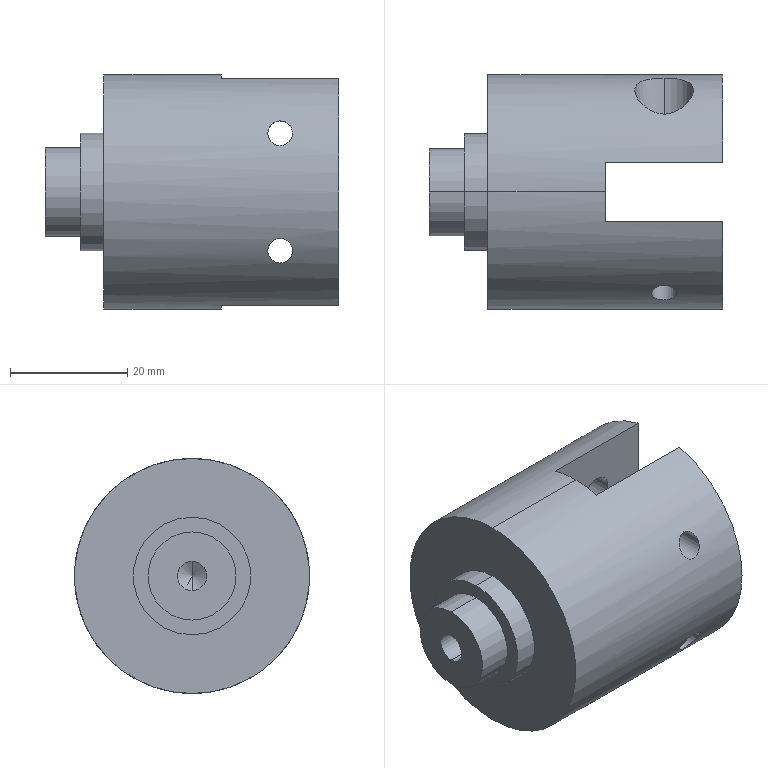Component | SolidWorks | RotationAxis-1 | 1 solid | 32 faces | box 50 x 40.01 x 40 mm | volume 42673 mm3 | cylinder 20 | plane 10 | cone 2 | commonest cylinder face diameters 10 x4 5.5 x4 4.2 x4 5 x2 15 x2 20 x2 40 x2
build123d program:
from build123d import *

# Parameters (mm, degrees)
SKETCH2_R                  = 20
BOSS_EXTRUDE1_DEPTH        = 40
SKETCH3_W                  = 54.214
SKETCH3_H                  = 10
CUT_EXTRUDE1_DEPTH         = 20
SKETCH4_R                  = 10
BOSS_EXTRUDE2_DEPTH        = 4
SKETCH6_R                  = 7.5
BOSS_EXTRUDE3_DEPTH        = 6
M6_TAPPED_HOLE1_D          = 5
M6_TAPPED_HOLE1_DEPTH      = 15
M6_TAPPED_HOLE1_TIP        = 1.502
SKETCH14_W                 = 2.1
SKETCH14_H                 = 15
M5_TAPPED_HOLE1_AT_2_COUNT = 2
M5_TAPPED_HOLE1_AT_2_PITCH = 20
SKETCH16_R                 = 2.75
CUT_EXTRUDE2_DEPTH         = 5
SKETCH17_R                 = 5
CUT_EXTRUDE3_DEPTH         = 12


with BuildPart() as part:
    # Sketch2 → Boss-Extrude1 (new body)
    with BuildSketch(Plane.XY):
        Circle(SKETCH2_R)
    extrude(amount=BOSS_EXTRUDE1_DEPTH)

    # Sketch3 → Cut-Extrude1 (cut)
    with BuildSketch(Plane(origin=(0, 0, 0), x_dir=(-1, 0, 0), z_dir=(0, 0, -1))):
        Rectangle(SKETCH3_W, SKETCH3_H)
    extrude(amount=-CUT_EXTRUDE1_DEPTH, mode=Mode.SUBTRACT)

    # Sketch4 → Boss-Extrude2 (add)
    with BuildSketch(Plane.XY.offset(40)):
        Circle(SKETCH4_R)
    extrude(amount=BOSS_EXTRUDE2_DEPTH)

    # Sketch6 → Boss-Extrude3 (add)
    with BuildSketch(Plane.XY.offset(44)):
        Circle(SKETCH6_R)
    extrude(amount=BOSS_EXTRUDE3_DEPTH)

    # M6 Tapped Hole1
    with Locations(Plane.XY.offset(50)):
        with Locations((0, 0)):
            Hole(M6_TAPPED_HOLE1_D / 2, depth=M6_TAPPED_HOLE1_DEPTH)
            with Locations((0, 0, -(M6_TAPPED_HOLE1_DEPTH + M6_TAPPED_HOLE1_TIP / 2))):  # 118° drill point
                Cone(0, M6_TAPPED_HOLE1_D / 2, M6_TAPPED_HOLE1_TIP, mode=Mode.SUBTRACT)

    # Sketch14 → M5 Tapped Hole1 (revolve, cut)
    with BuildSketch(Plane(origin=(-10, -5, 10), x_dir=(0, 0, 1), z_dir=(1, 0, 0))):
        with Locations((1.05, 7.5)):
            Rectangle(SKETCH14_W, SKETCH14_H)
    m5_tapped_hole1 = revolve(axis=Axis((-10, 1.35, 10), (0, -1, 0)), mode=Mode.SUBTRACT)

    # M5 Tapped Hole1 at 2: M5 Tapped Hole1 ×2
    with Locations(*[(i * M5_TAPPED_HOLE1_AT_2_PITCH, 0, 0) for i in range(1, M5_TAPPED_HOLE1_AT_2_COUNT)]):
        add(m5_tapped_hole1, mode=Mode.SUBTRACT)

    # Sketch16 → Cut-Extrude2 (cut)
    with BuildSketch(Plane.XZ.offset(-5)):
        with Locations((-10, 10)):
            Circle(SKETCH16_R)
        with Locations((10, 10)):
            Circle(SKETCH16_R)
    extrude(amount=-CUT_EXTRUDE2_DEPTH, mode=Mode.SUBTRACT)

    # Sketch17 → Cut-Extrude3 (cut)
    with BuildSketch(Plane.XZ.offset(-10)):
        with Locations((-10, 10)):
            Circle(SKETCH17_R)
        with Locations((10, 10)):
            Circle(SKETCH17_R)
    extrude(amount=-CUT_EXTRUDE3_DEPTH, mode=Mode.SUBTRACT)


solid = part.part

# Placed as in the assembly
solid = solid.moved(Location((1592.163, 3833.699, 1079.241), (0, -90, 0)))